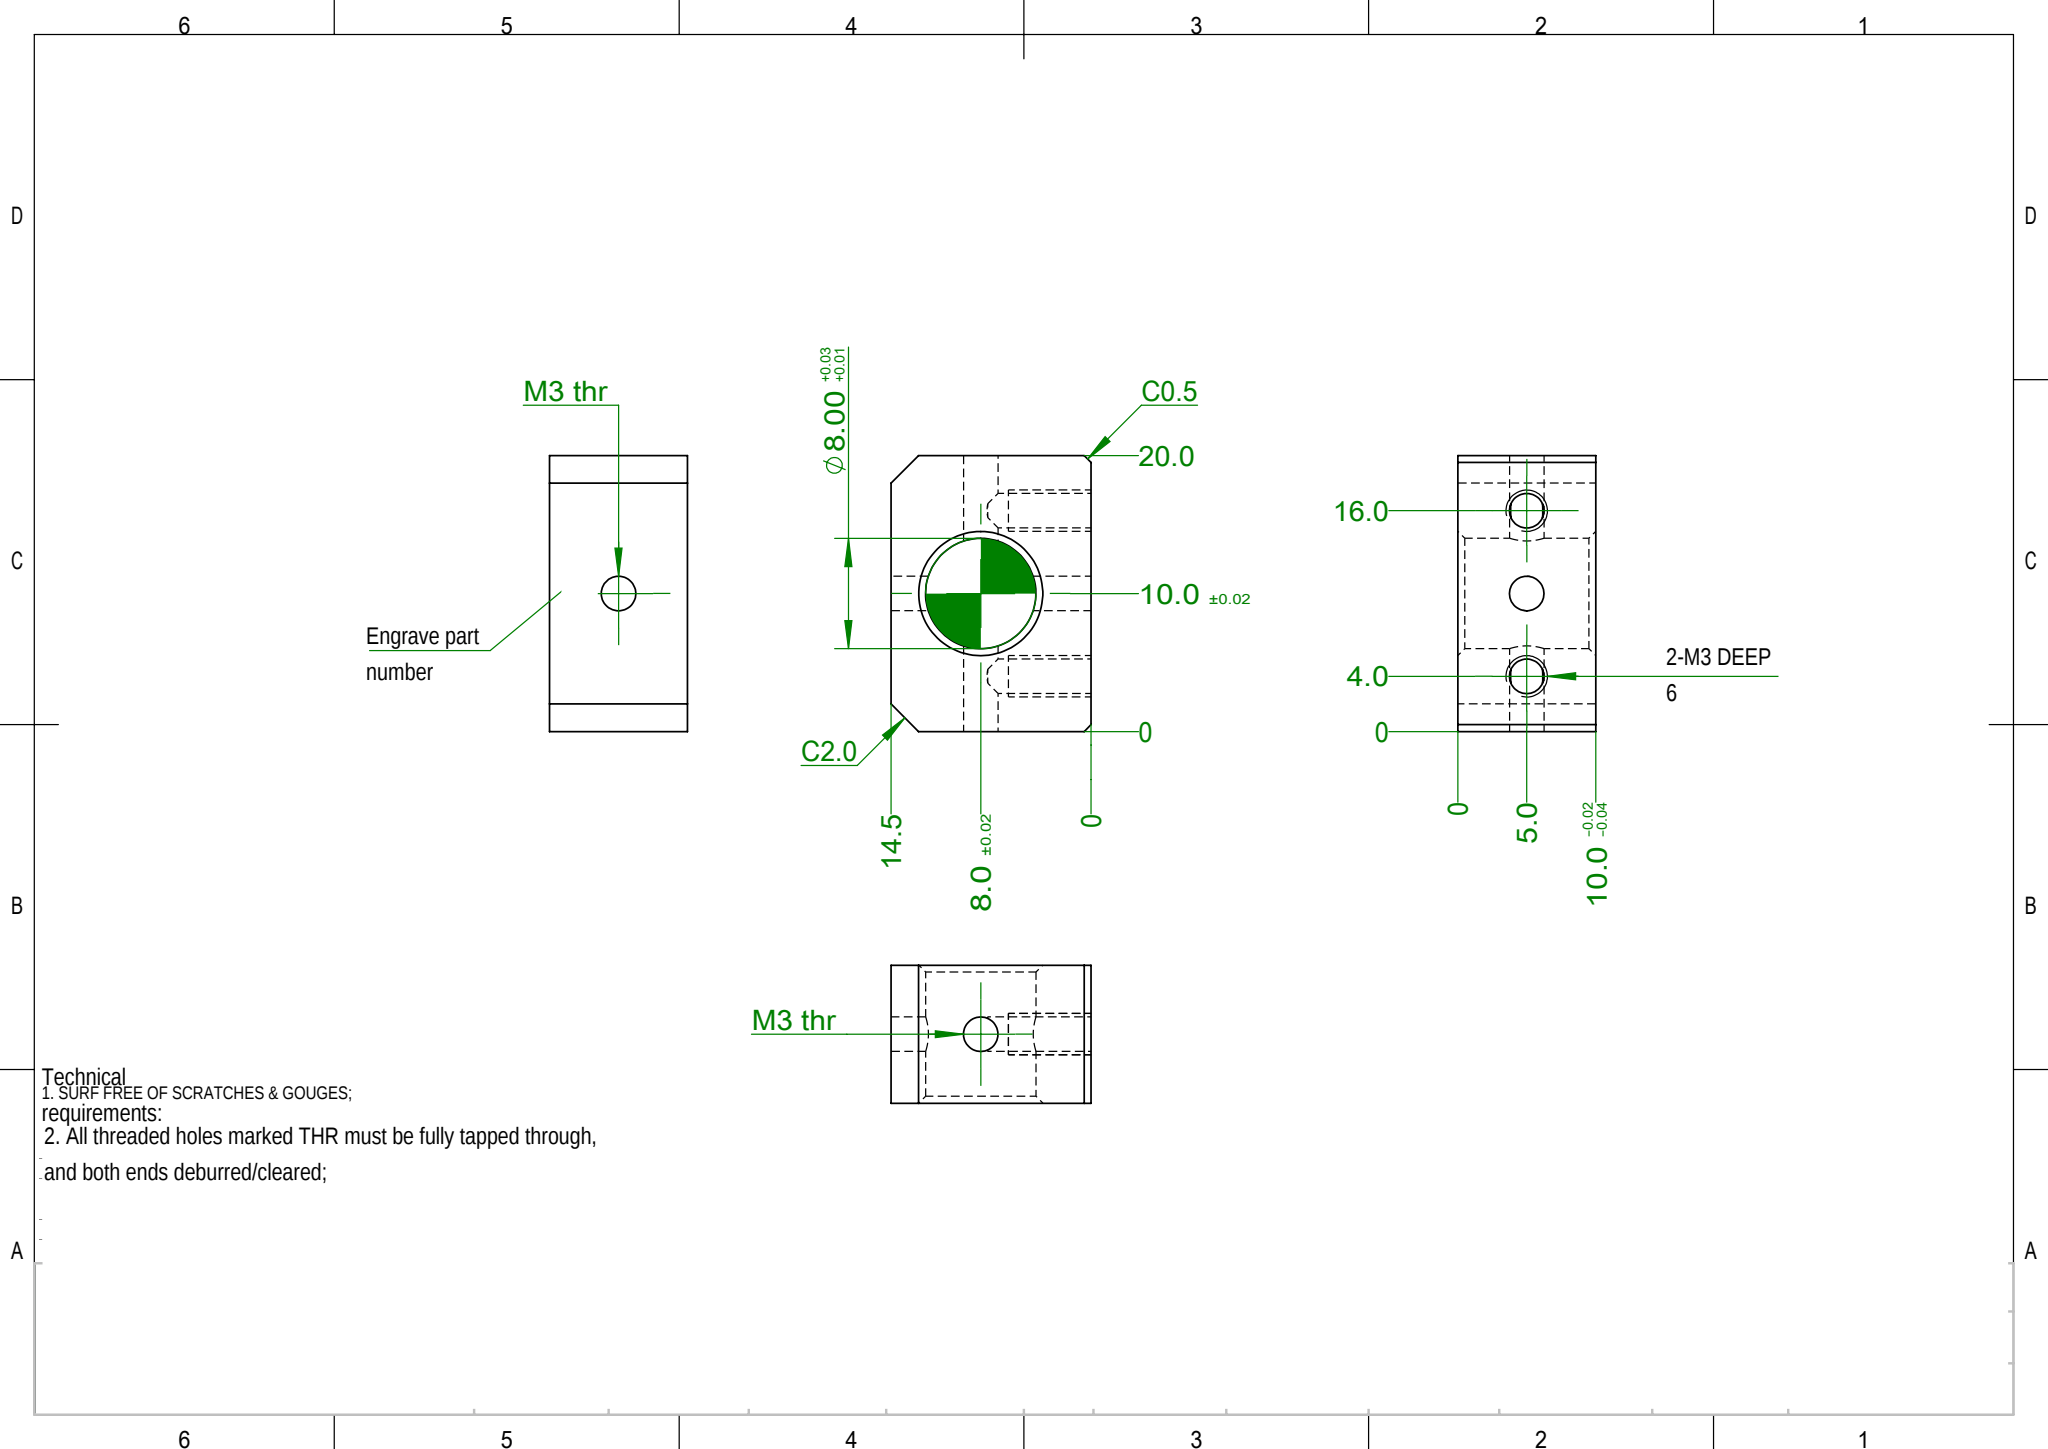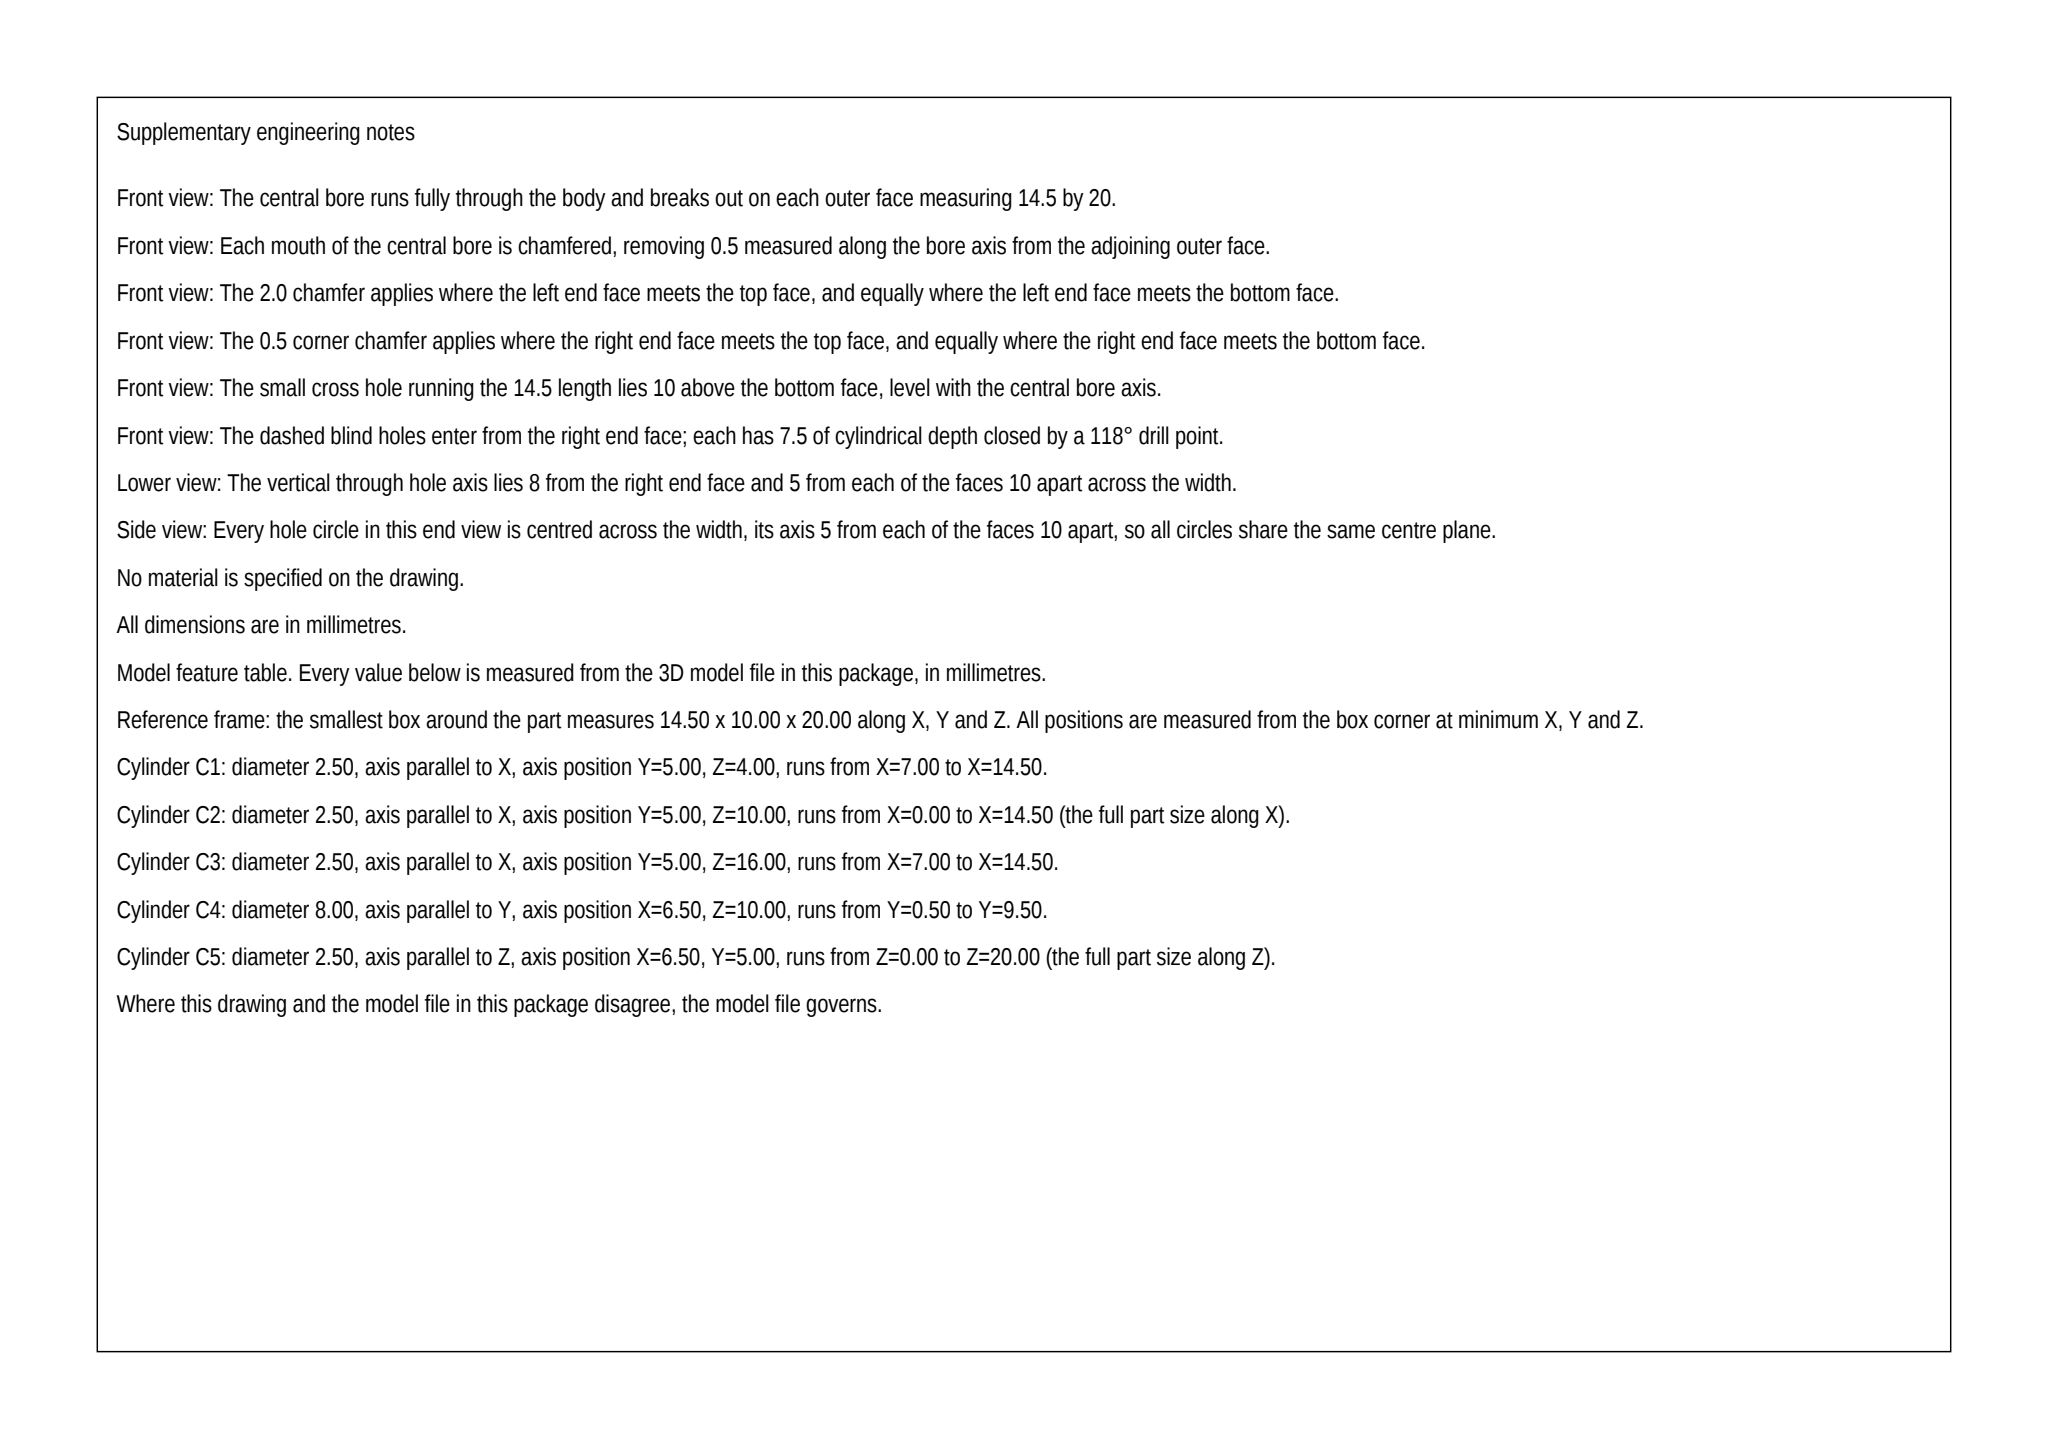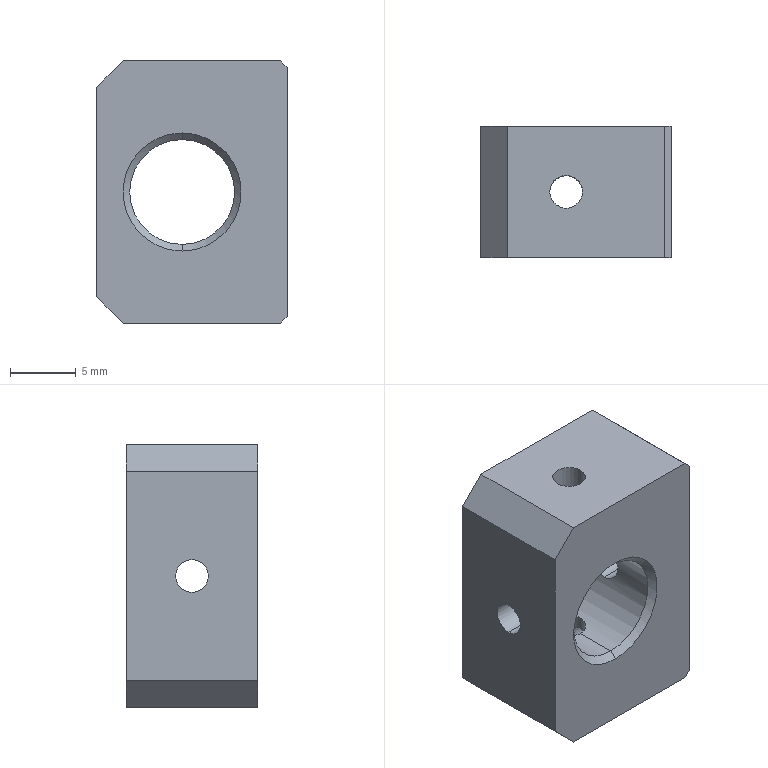Part | SolidWorks | mm | 1 solid | 32 faces | box 14.5 x 10 x 20 mm | volume 2188 mm3 | cylinder 14 | plane 10 | cone 8 | commonest cylinder face diameters 2.5 x12 8 x2
Drawing notes:
C2.0 CHAMFER 2X: UPPER & LOWER LEFT CORNERS, FRONT VIEW | from the solid: bbox 14.5 x 10.0 x 20.0; no fillet radii; symmetric chamfered corners at z=0 face ends x=0 and x=14.5, per C2.0 callout